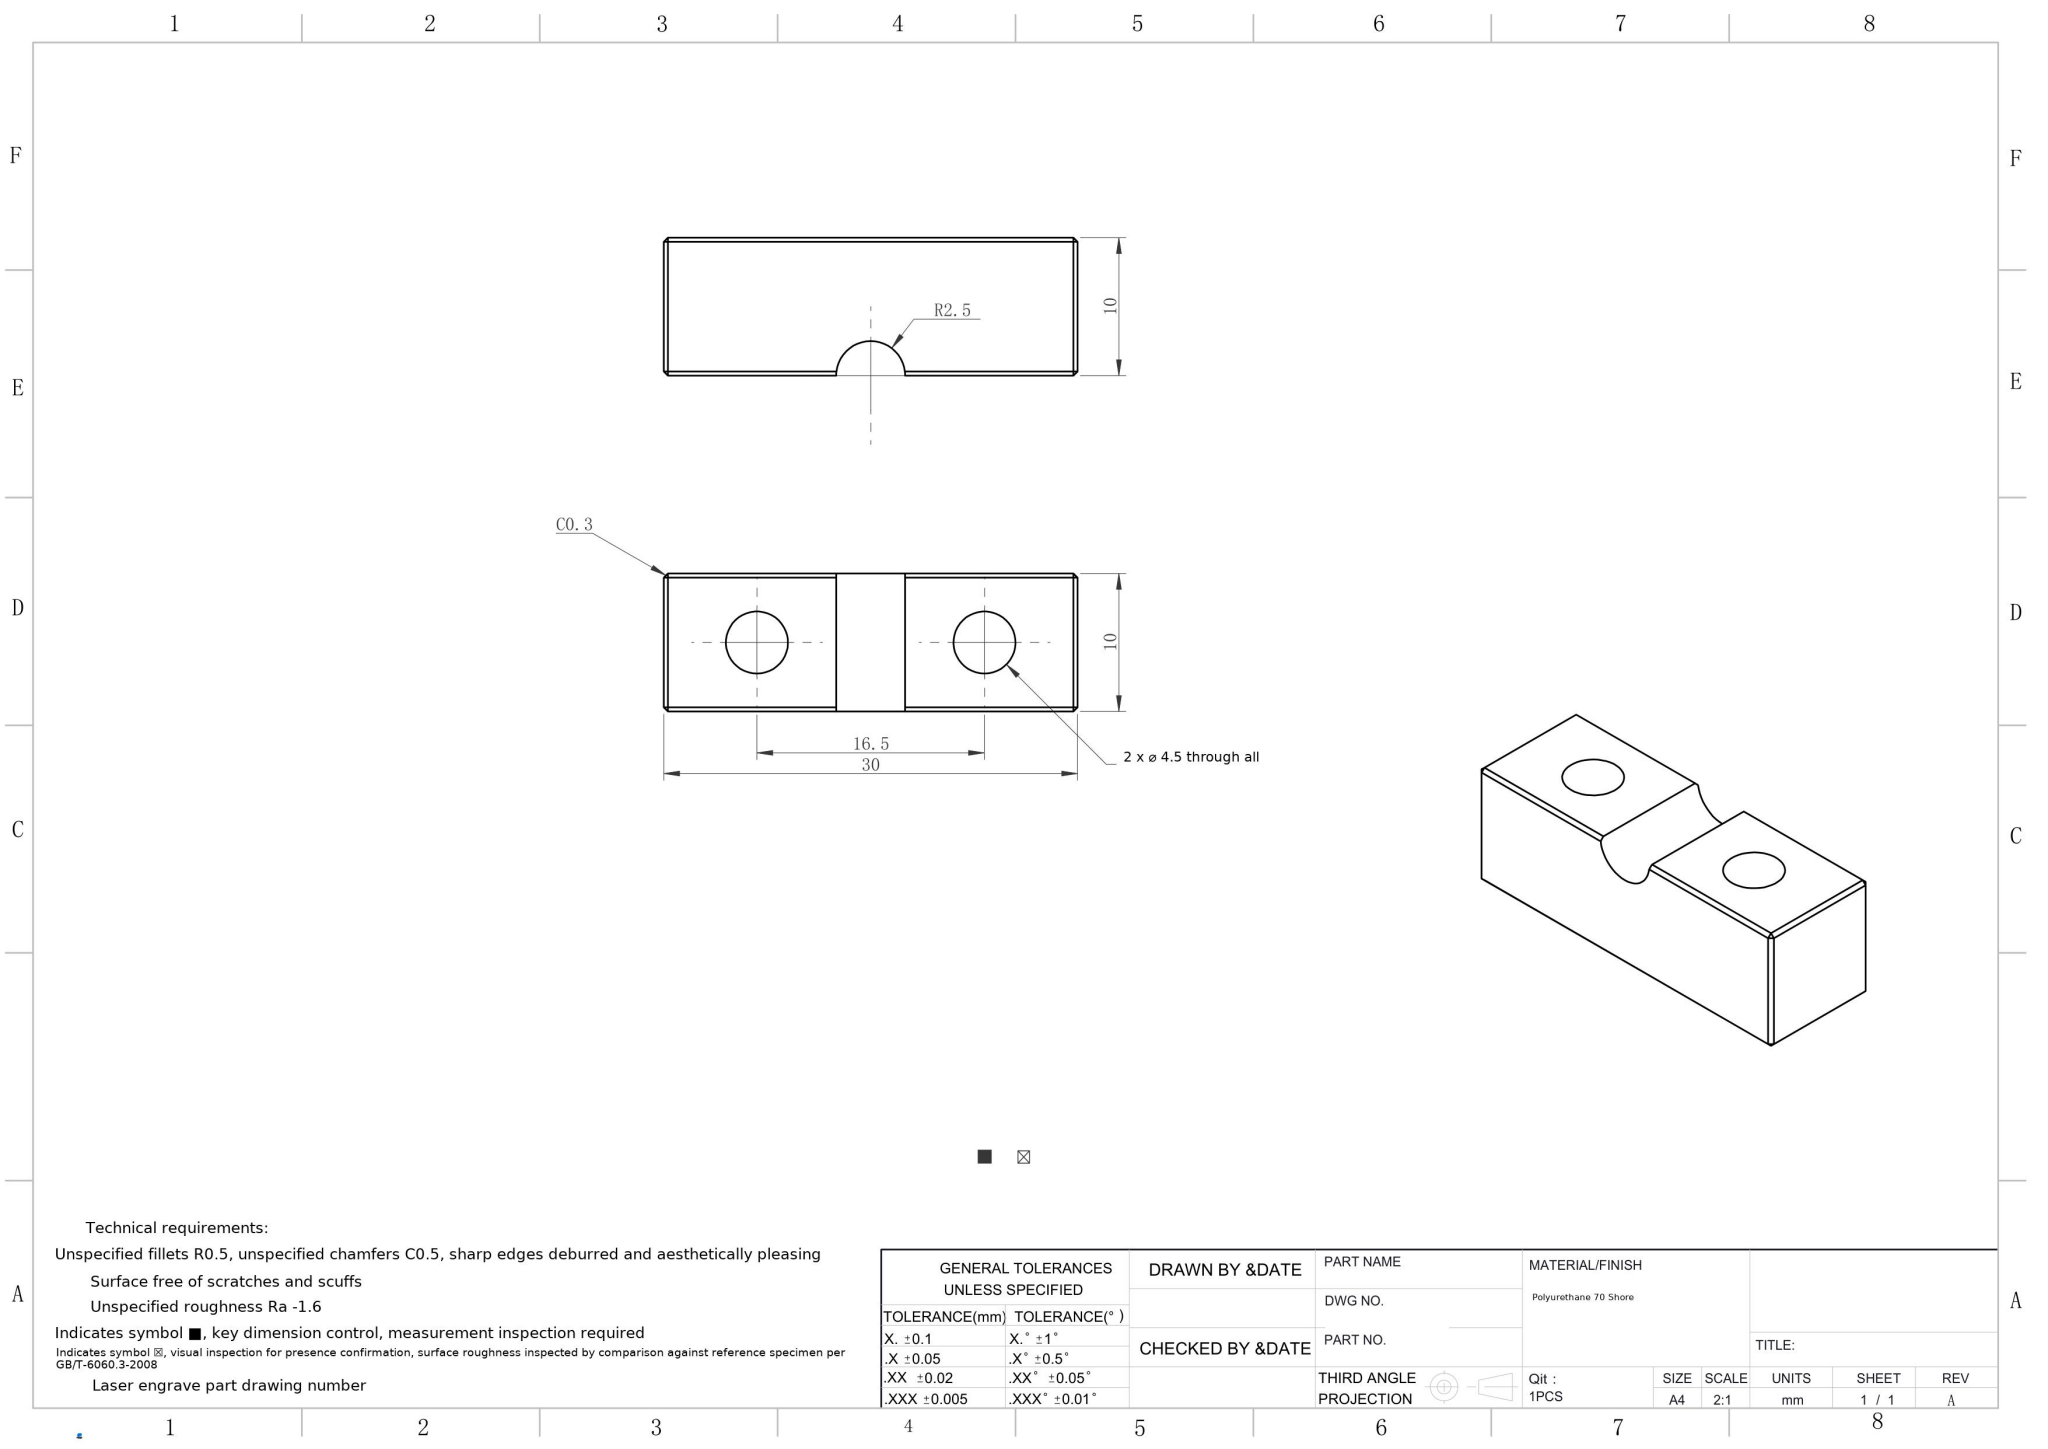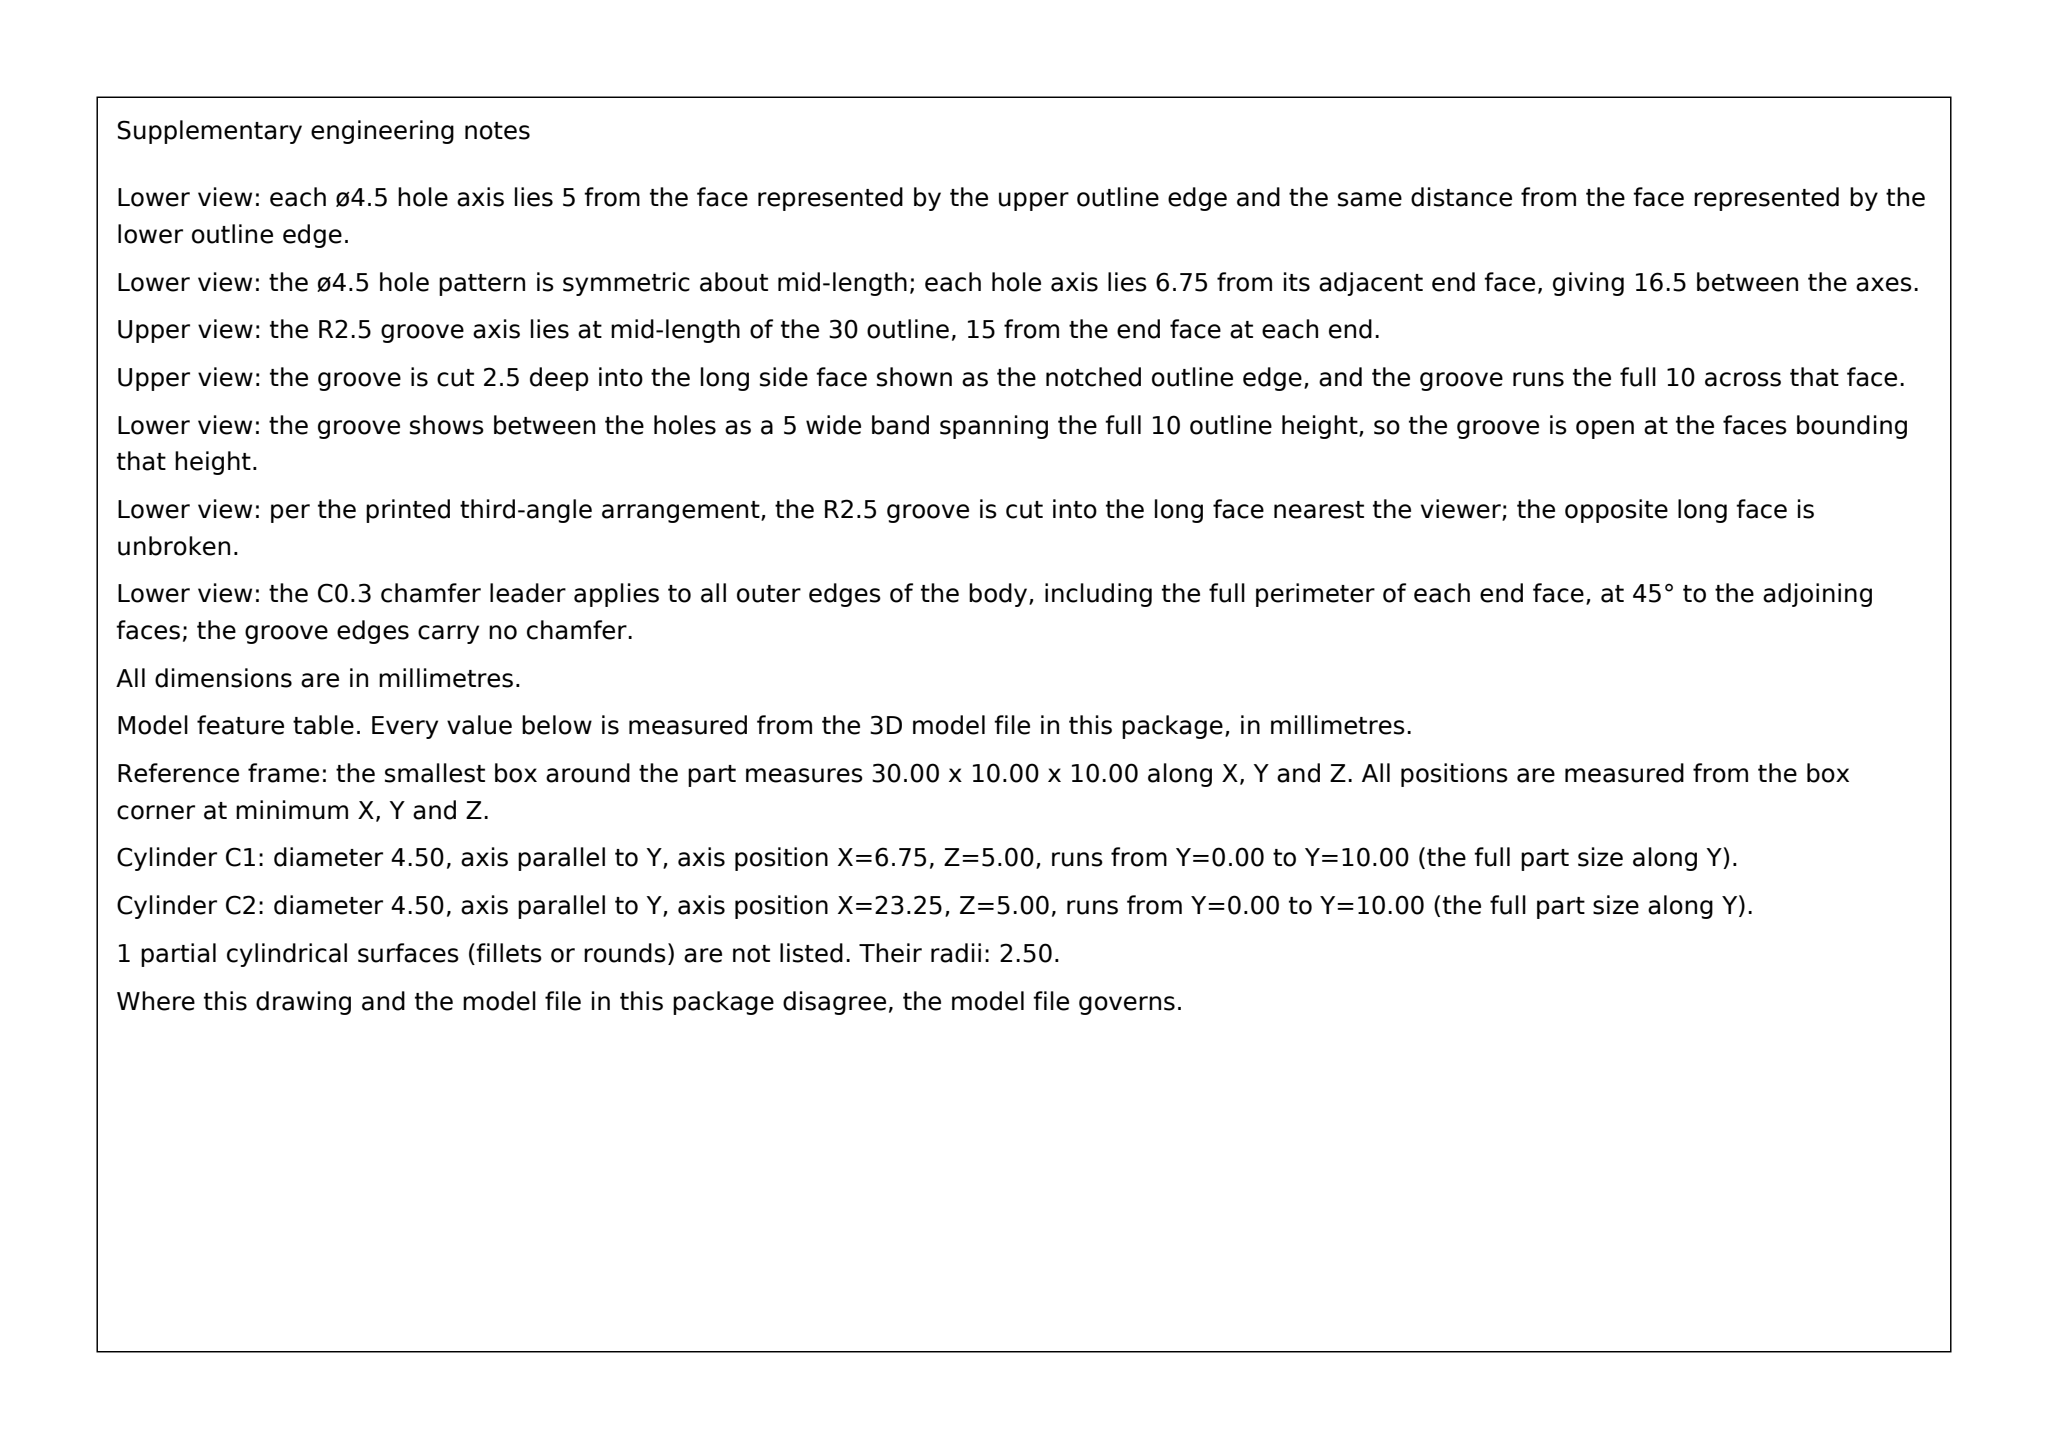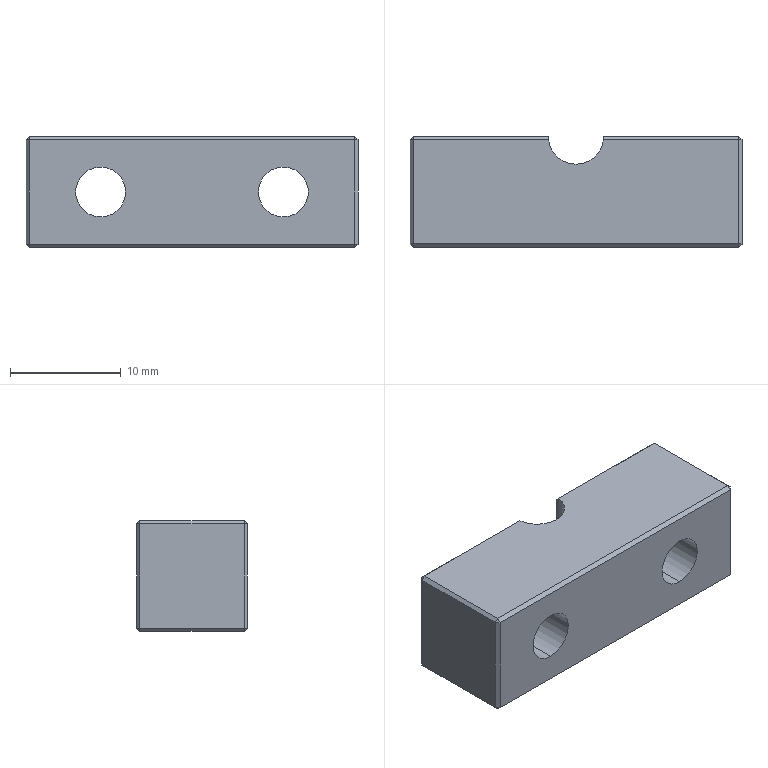Part | SolidWorks | mm | material Polyurethane 70 Shore | 1 solid | 34 faces | box 30 x 10 x 10 mm | volume 2575 mm3 | plane 29 | cylinder 5 | commonest cylinder face diameters 4.5 x4 5 x1
Drawing notes:
2X Ø4.5 THRU, hole axes 5 from bottom face and 5 from front face; located 6.75 and 23.25 from left end face | from the solid: cylinders [4.5,'y',[6.75,null,5.0],10.0] and [4.5,'y',[23.25,null,5.0],10.0]; bbox 30x10x10
R2.5 semicircular notch (Ø5 through 10 thickness) centered 15 from left end face, open to top face | from the solid: cylinder [5.0,'z',[15.0,10.0,null],10.0]; axis planes x=0/x=30, y=10
2X Ø4.5 THRU, hole axes 5 from bottom face and 5 from front face, located 6.75 and 23.25 from left end face | from the solid: cylinders[dia 4.5, axis y, pos (6.75,-,5.0) and (23.25,-,5.0), length 10]
build123d program:
from build123d import *

# Parameters (mm, degrees)
SKETCH1_W            = 30
SKETCH1_H            = 10
BOSS_EXTRUDE1_DEPTH  = 10
SKETCH2_R            = 2.5
CUT_EXTRUDE1_DEPTH   = 19.708
M4_CLEARANCE_HOLE1_D = 4.5
CHAMFER1_SIZE        = 0.3


with BuildPart() as part:
    # Sketch1 → Boss-Extrude1 (new body)
    with BuildSketch(Plane.XY):
        Rectangle(SKETCH1_W, SKETCH1_H)
    extrude(amount=BOSS_EXTRUDE1_DEPTH)

    # Sketch2 → Cut-Extrude1 (cut, through all)
    with BuildSketch(Plane.XY.offset(10)):
        with Locations((0, 5)):
            Circle(SKETCH2_R)
    extrude(amount=-CUT_EXTRUDE1_DEPTH, mode=Mode.SUBTRACT)

    # M4 Clearance Hole1 (through all)
    with Locations(Plane(origin=(0, 5, 0), x_dir=(1, 0, 0), z_dir=(0, 1, 0))):
        with Locations((8.25, -5), (-8.25, -5)):
            Hole(M4_CLEARANCE_HOLE1_D / 2)

    # Chamfer1
    chamfer1_edges = [part.edges().sort_by_distance(p)[0] for p in [
        (-15, 0, 10),
        (-8.75, 5, 0),
        (-8.75, 5, 10),
        (0, -5, 10),
        (15, 0, 10),
        (0, -5, 0),
        (-15, 0, 0),
        (8.75, 5, 0),
        (15, 0, 0),
        (15, -5, 5),
        (-15, -5, 5),
        (-15, 5, 5),
        (15, 5, 5),
        (8.75, 5, 10),
    ]]
    chamfer(chamfer1_edges, length=CHAMFER1_SIZE)


solid = part.part